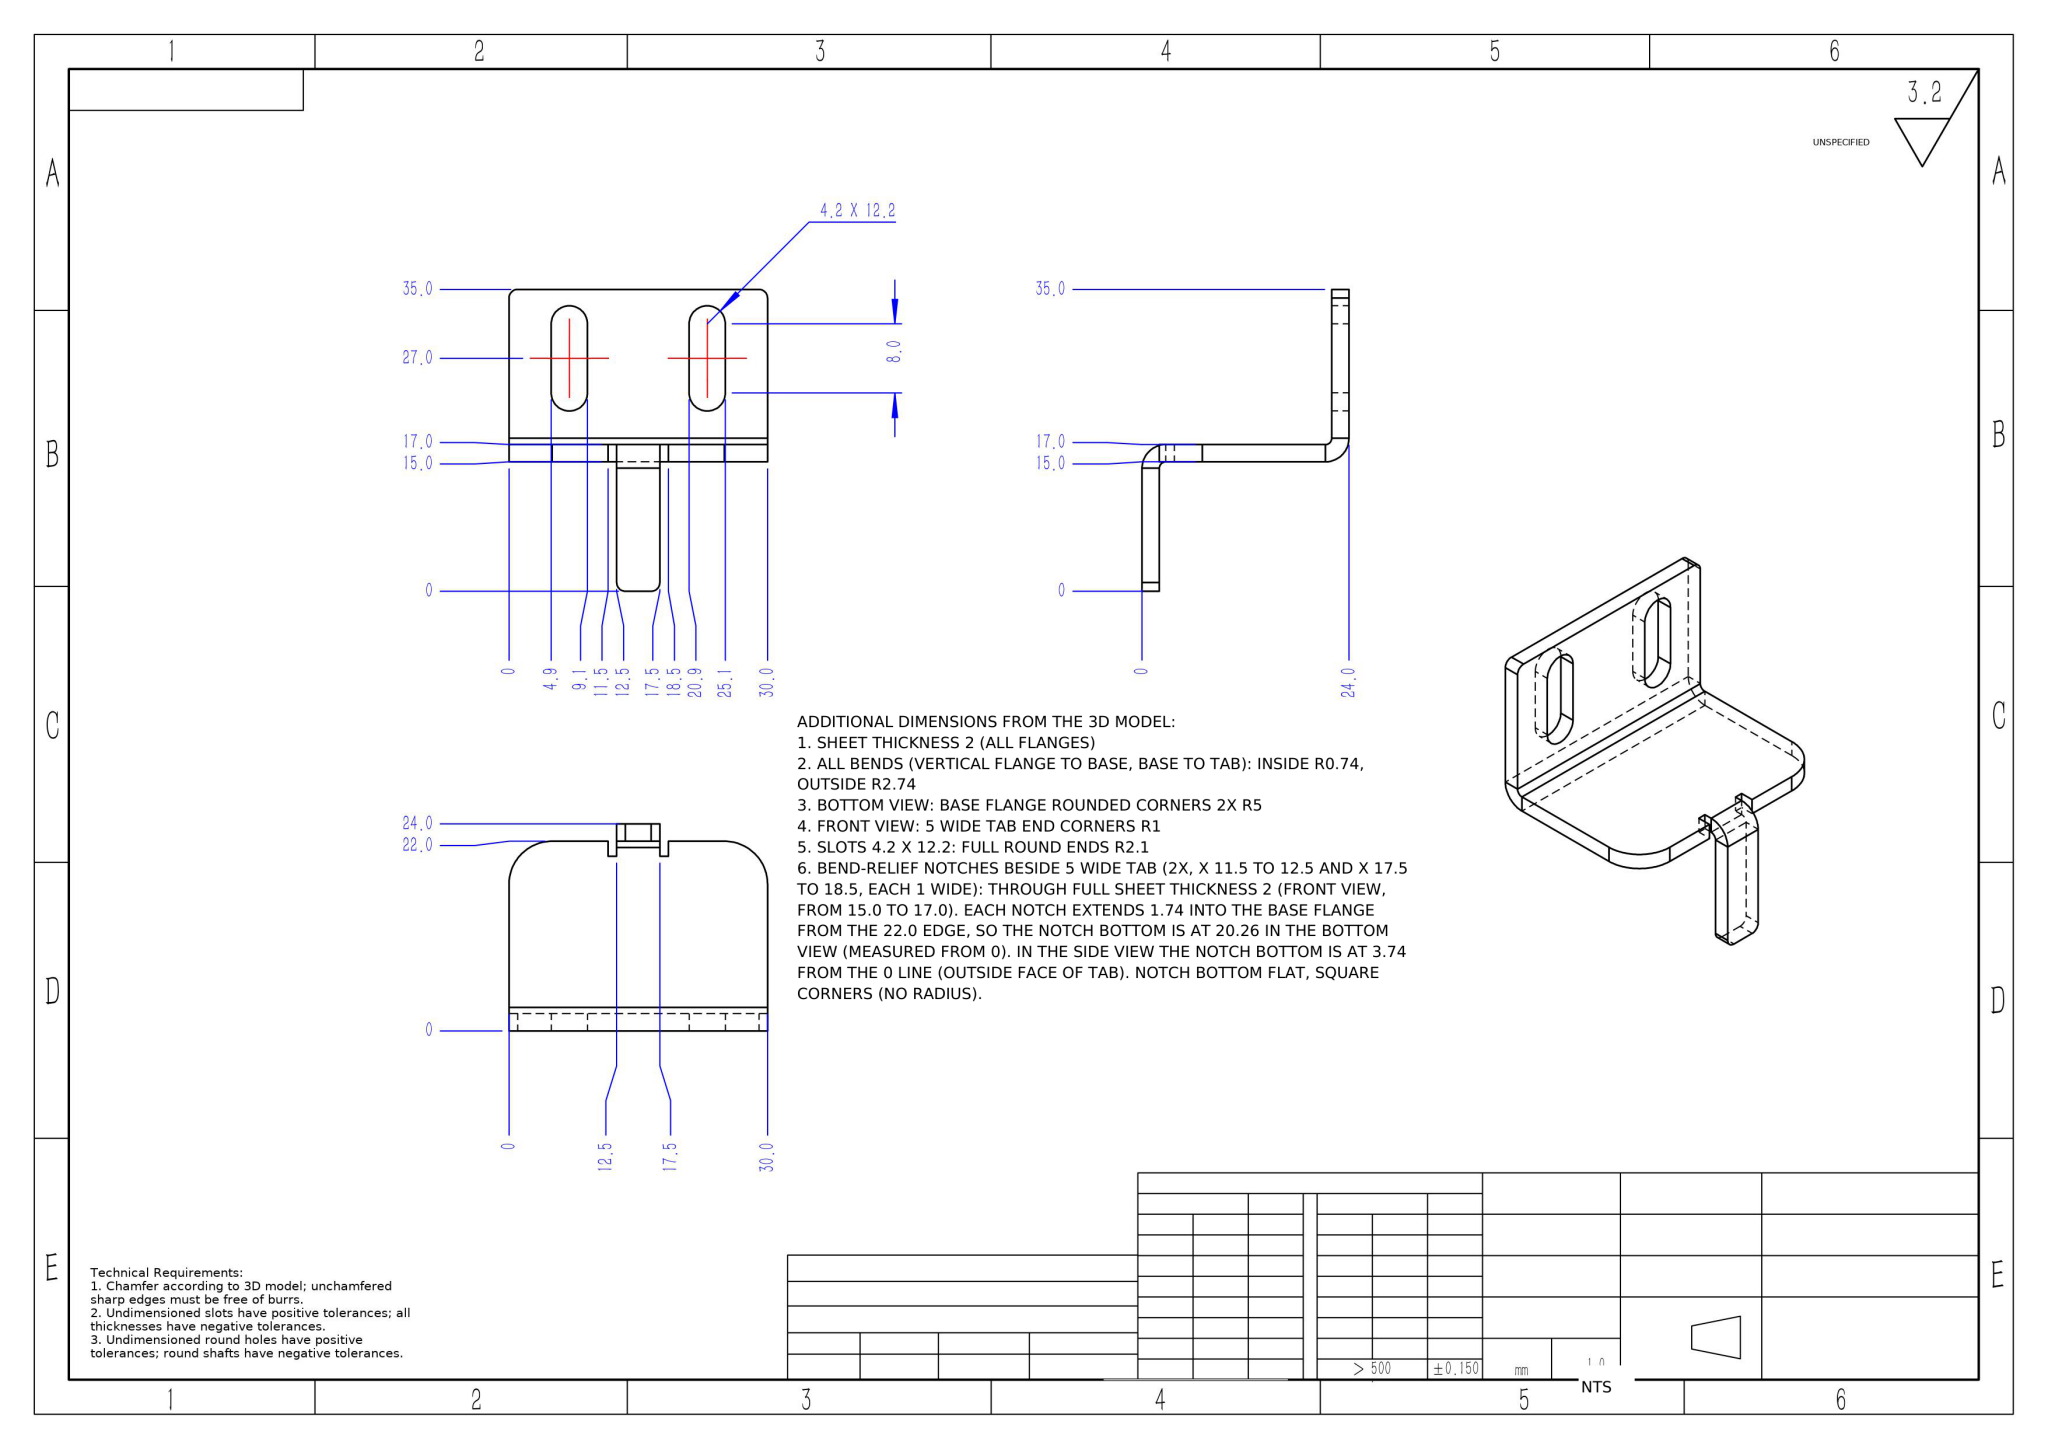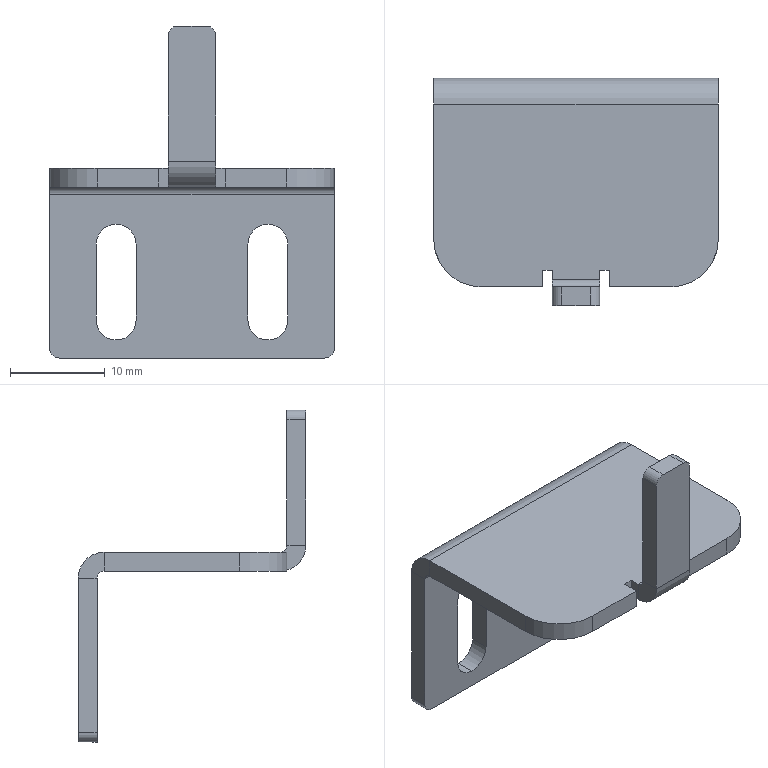Part | NX | mm | 1 solid | 46 faces | box 30 x 24 x 35 mm | volume 2298 mm3 | plane 30 | cylinder 16 | commonest cylinder face diameters 4.2 x6 2 x4 5.473 x2 1.473 x2 10 x2